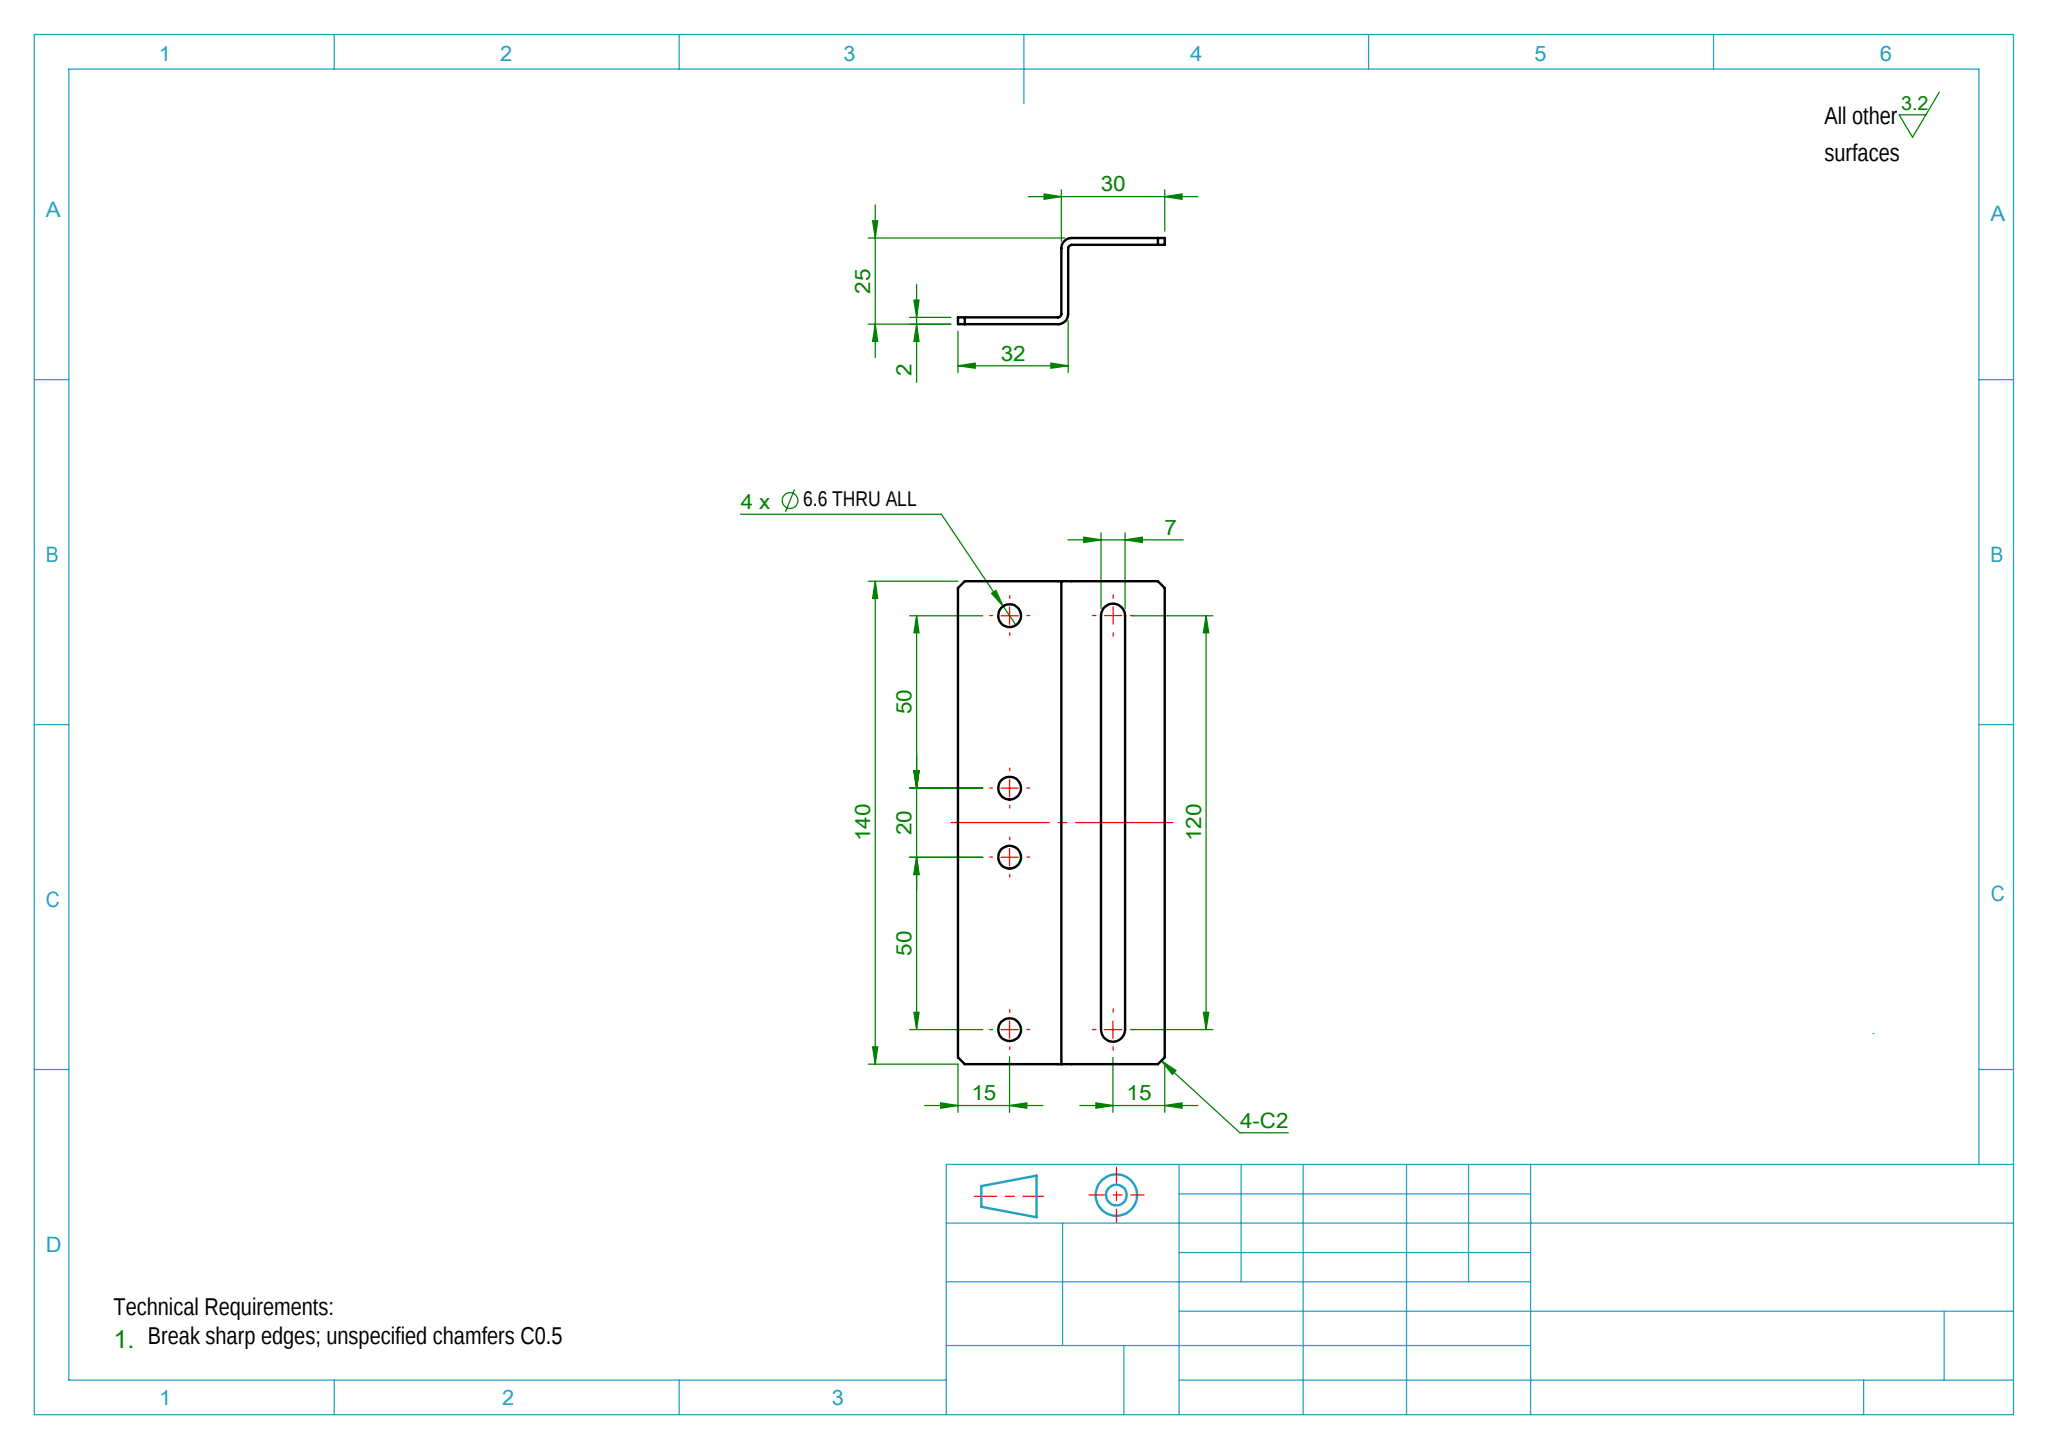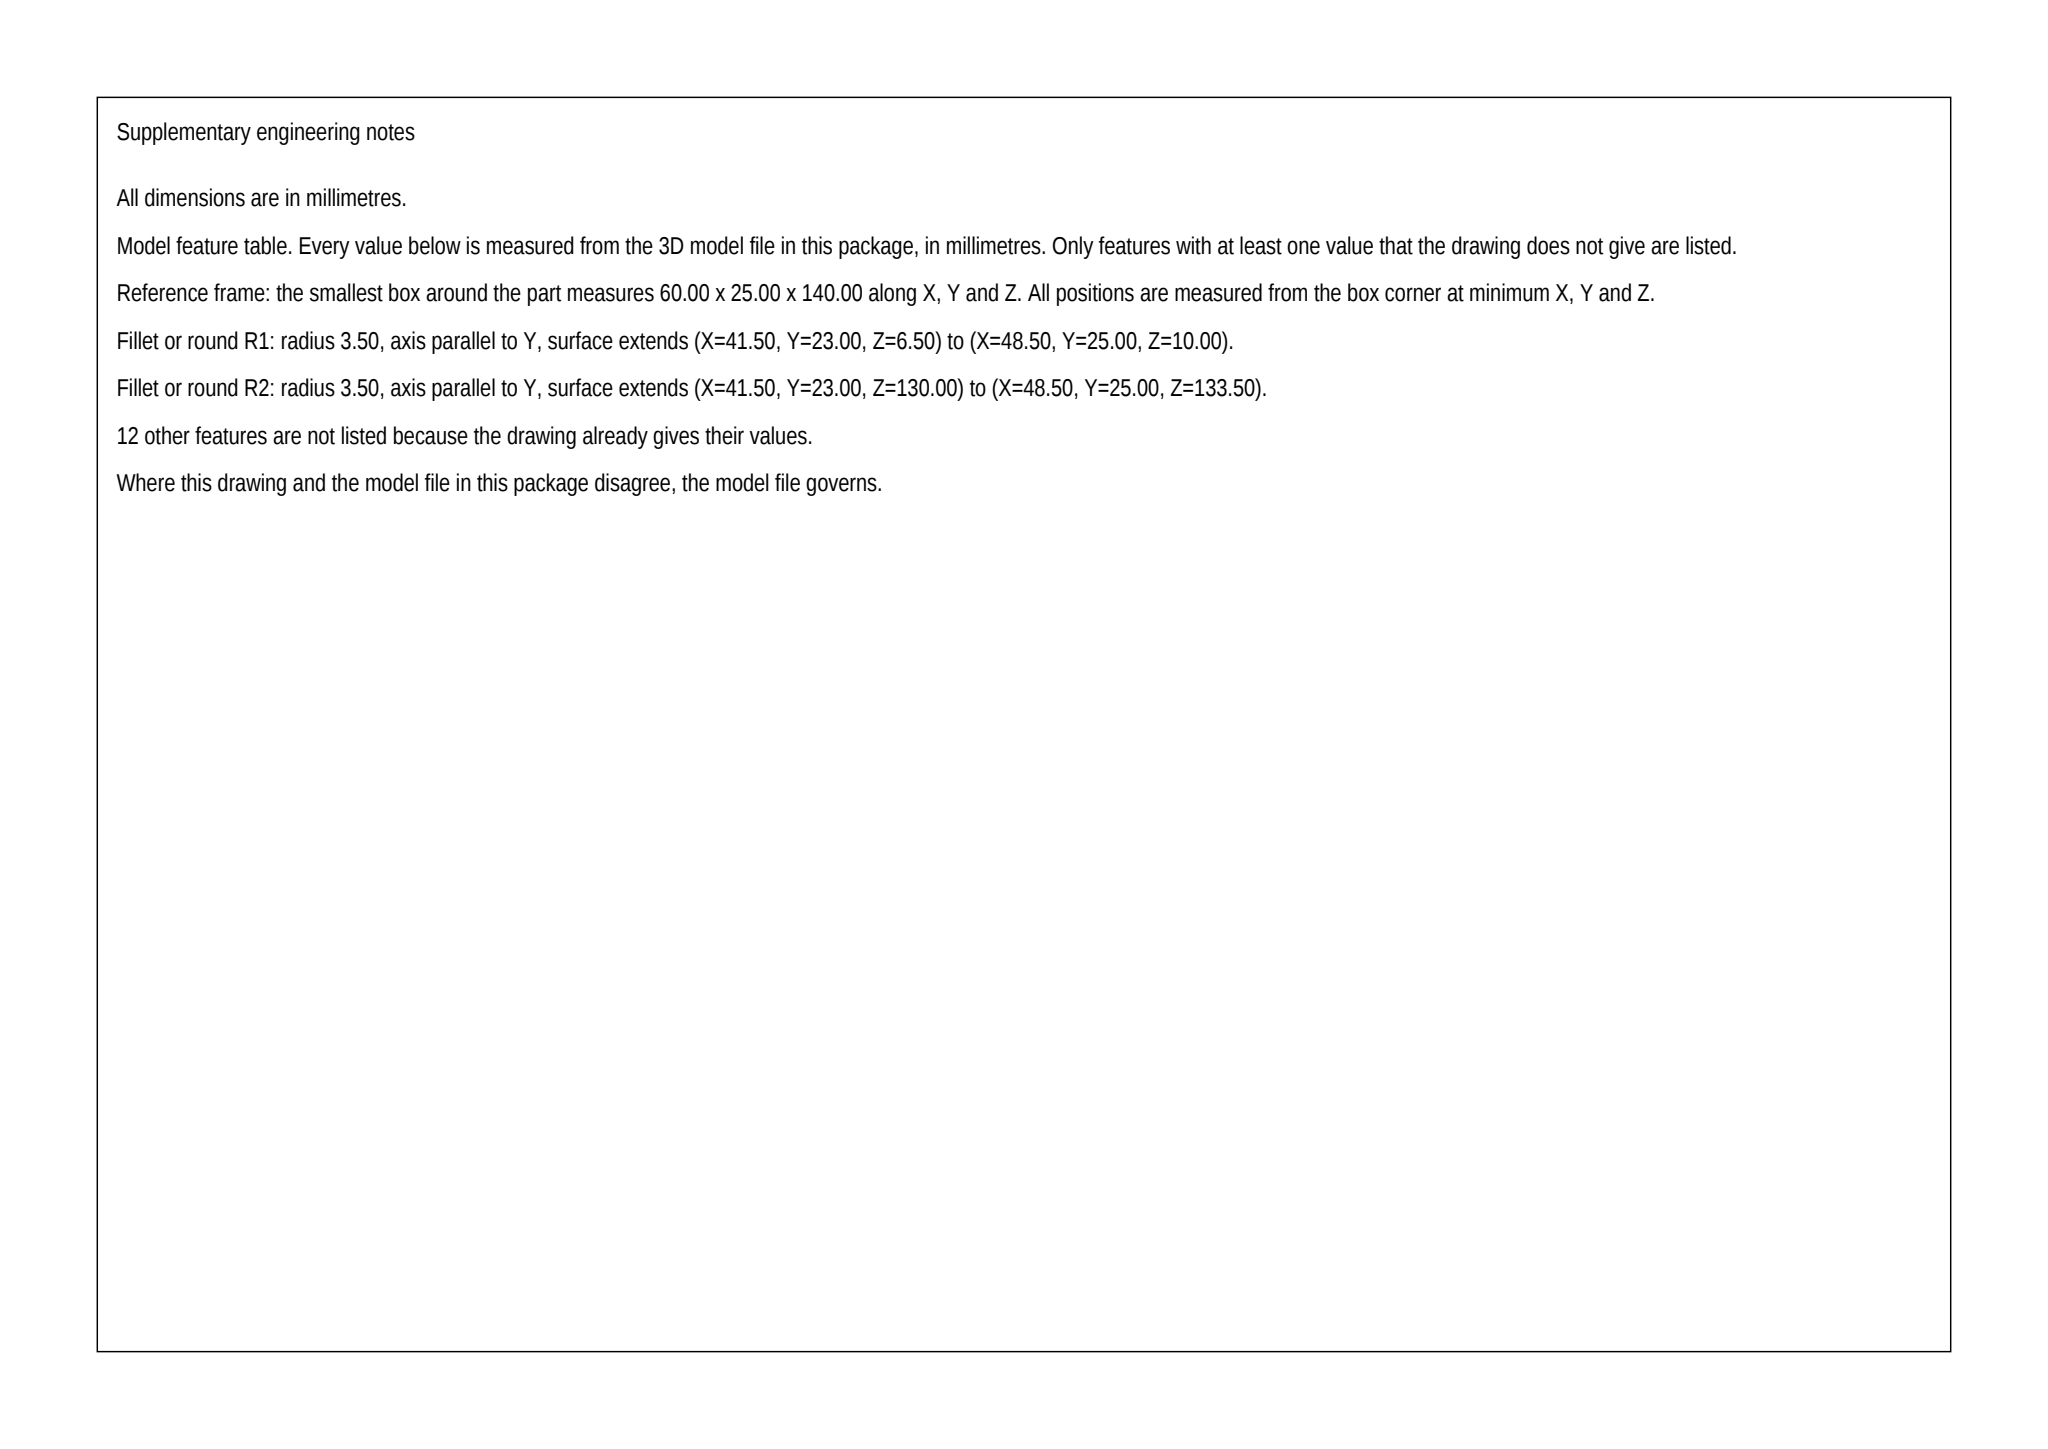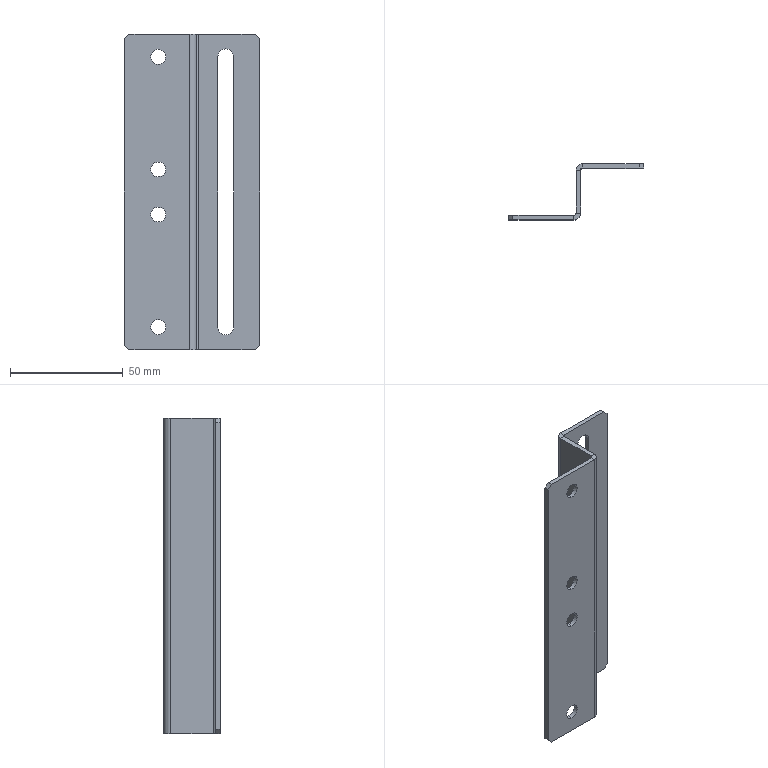Part | SolidWorks | mm | 1 solid | 39 faces | box 60 x 25 x 140 mm | volume 20713 mm3 | plane 24 | cylinder 15 | commonest cylinder face diameters 6.6 x8 7 x3 6 x2 2 x2